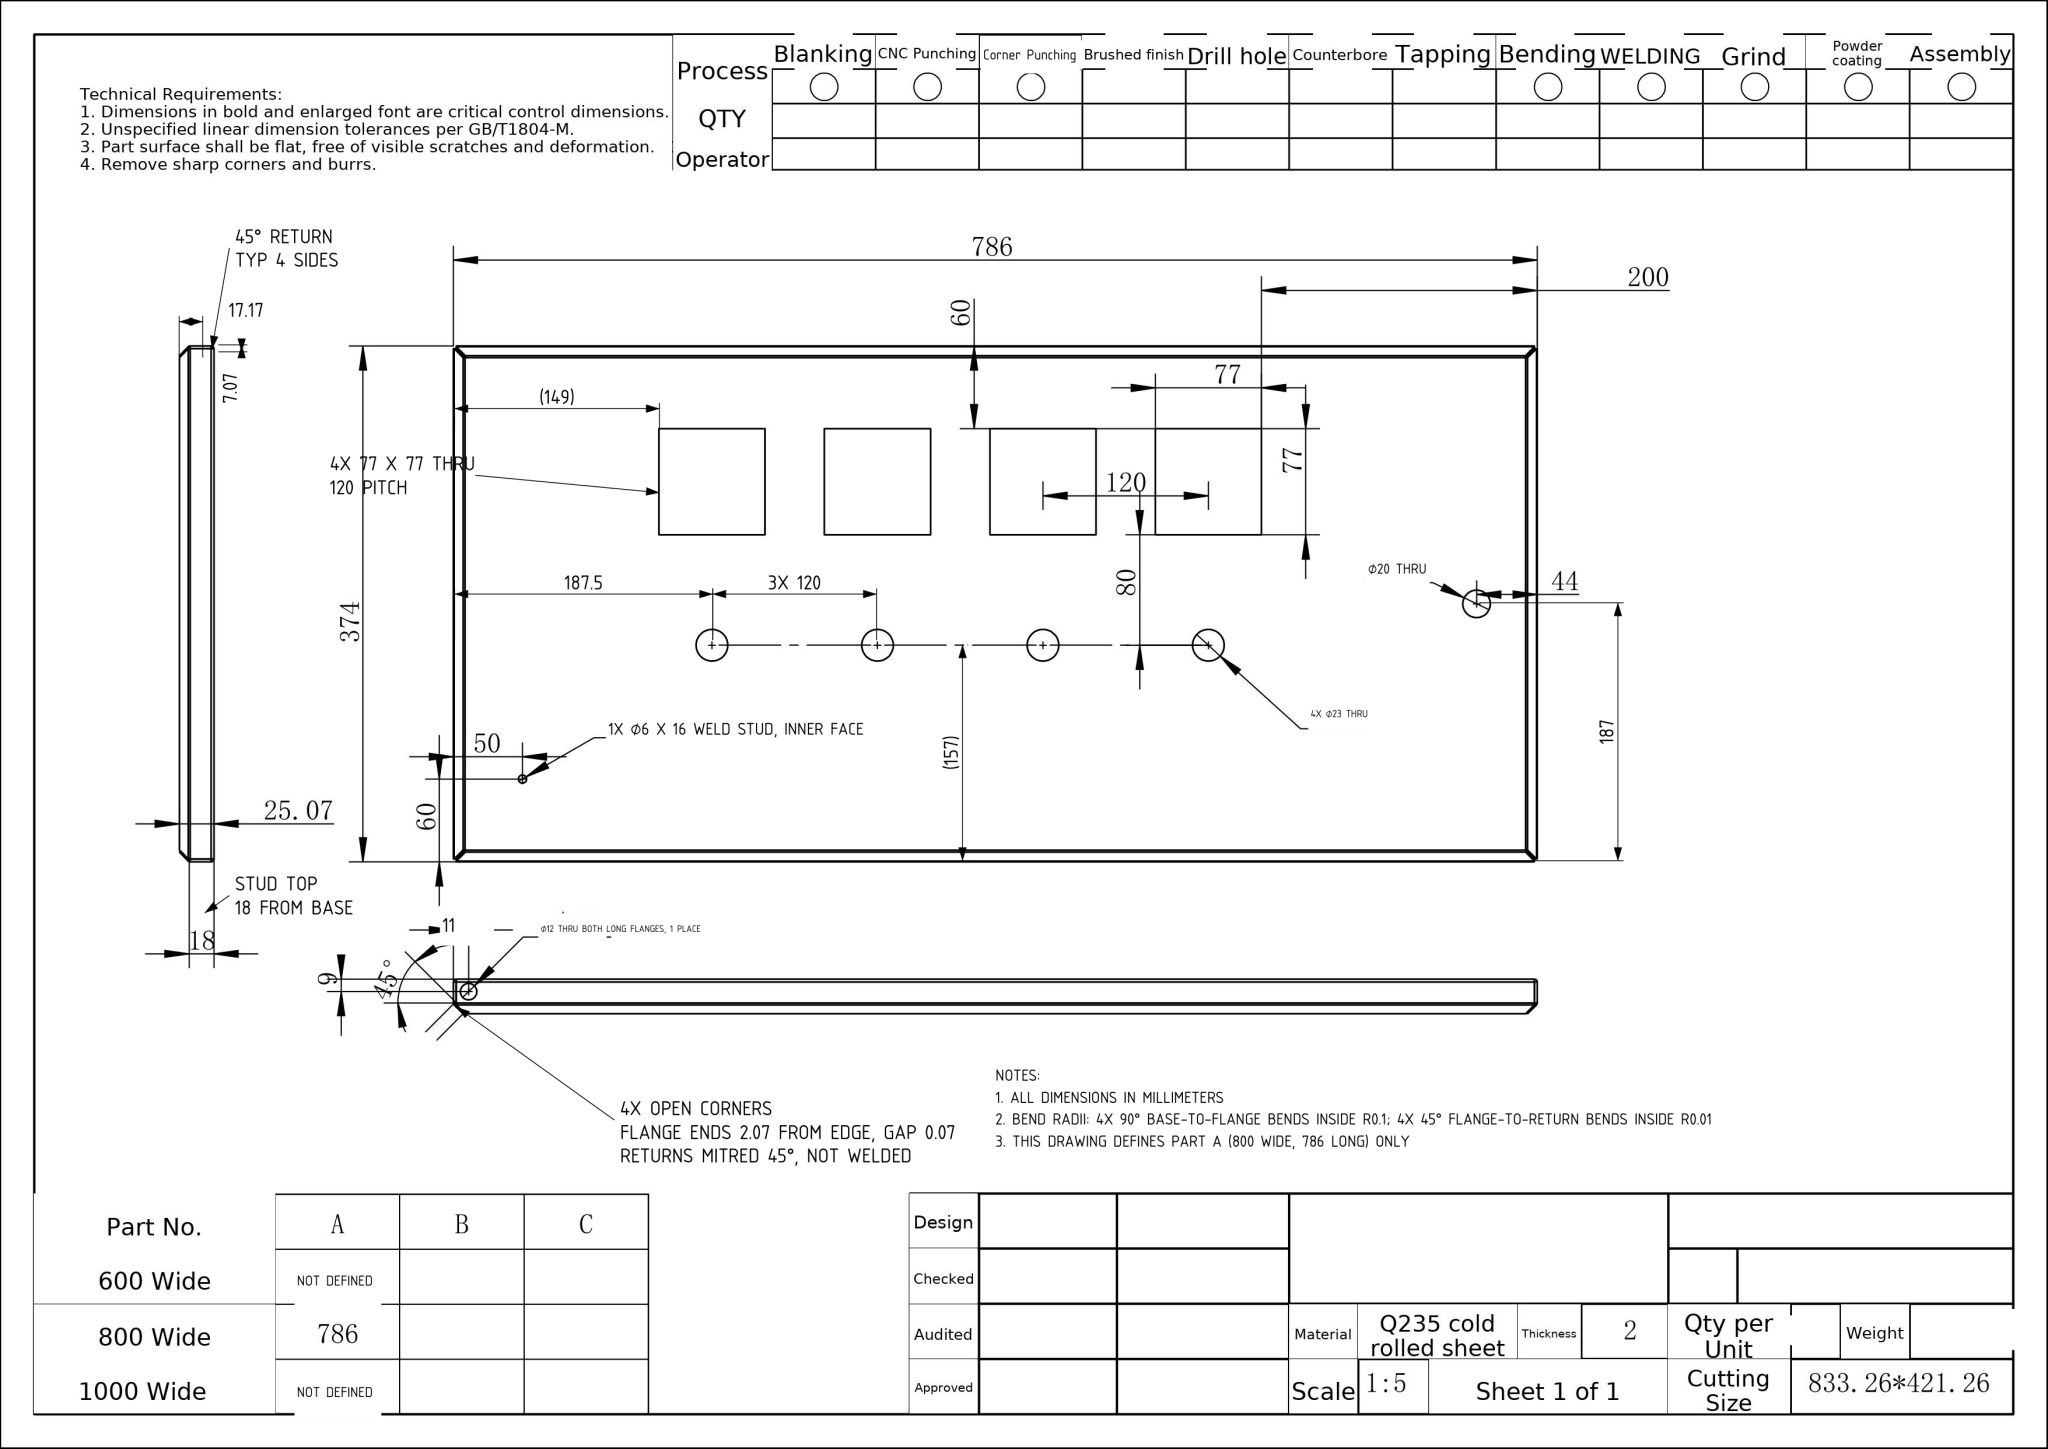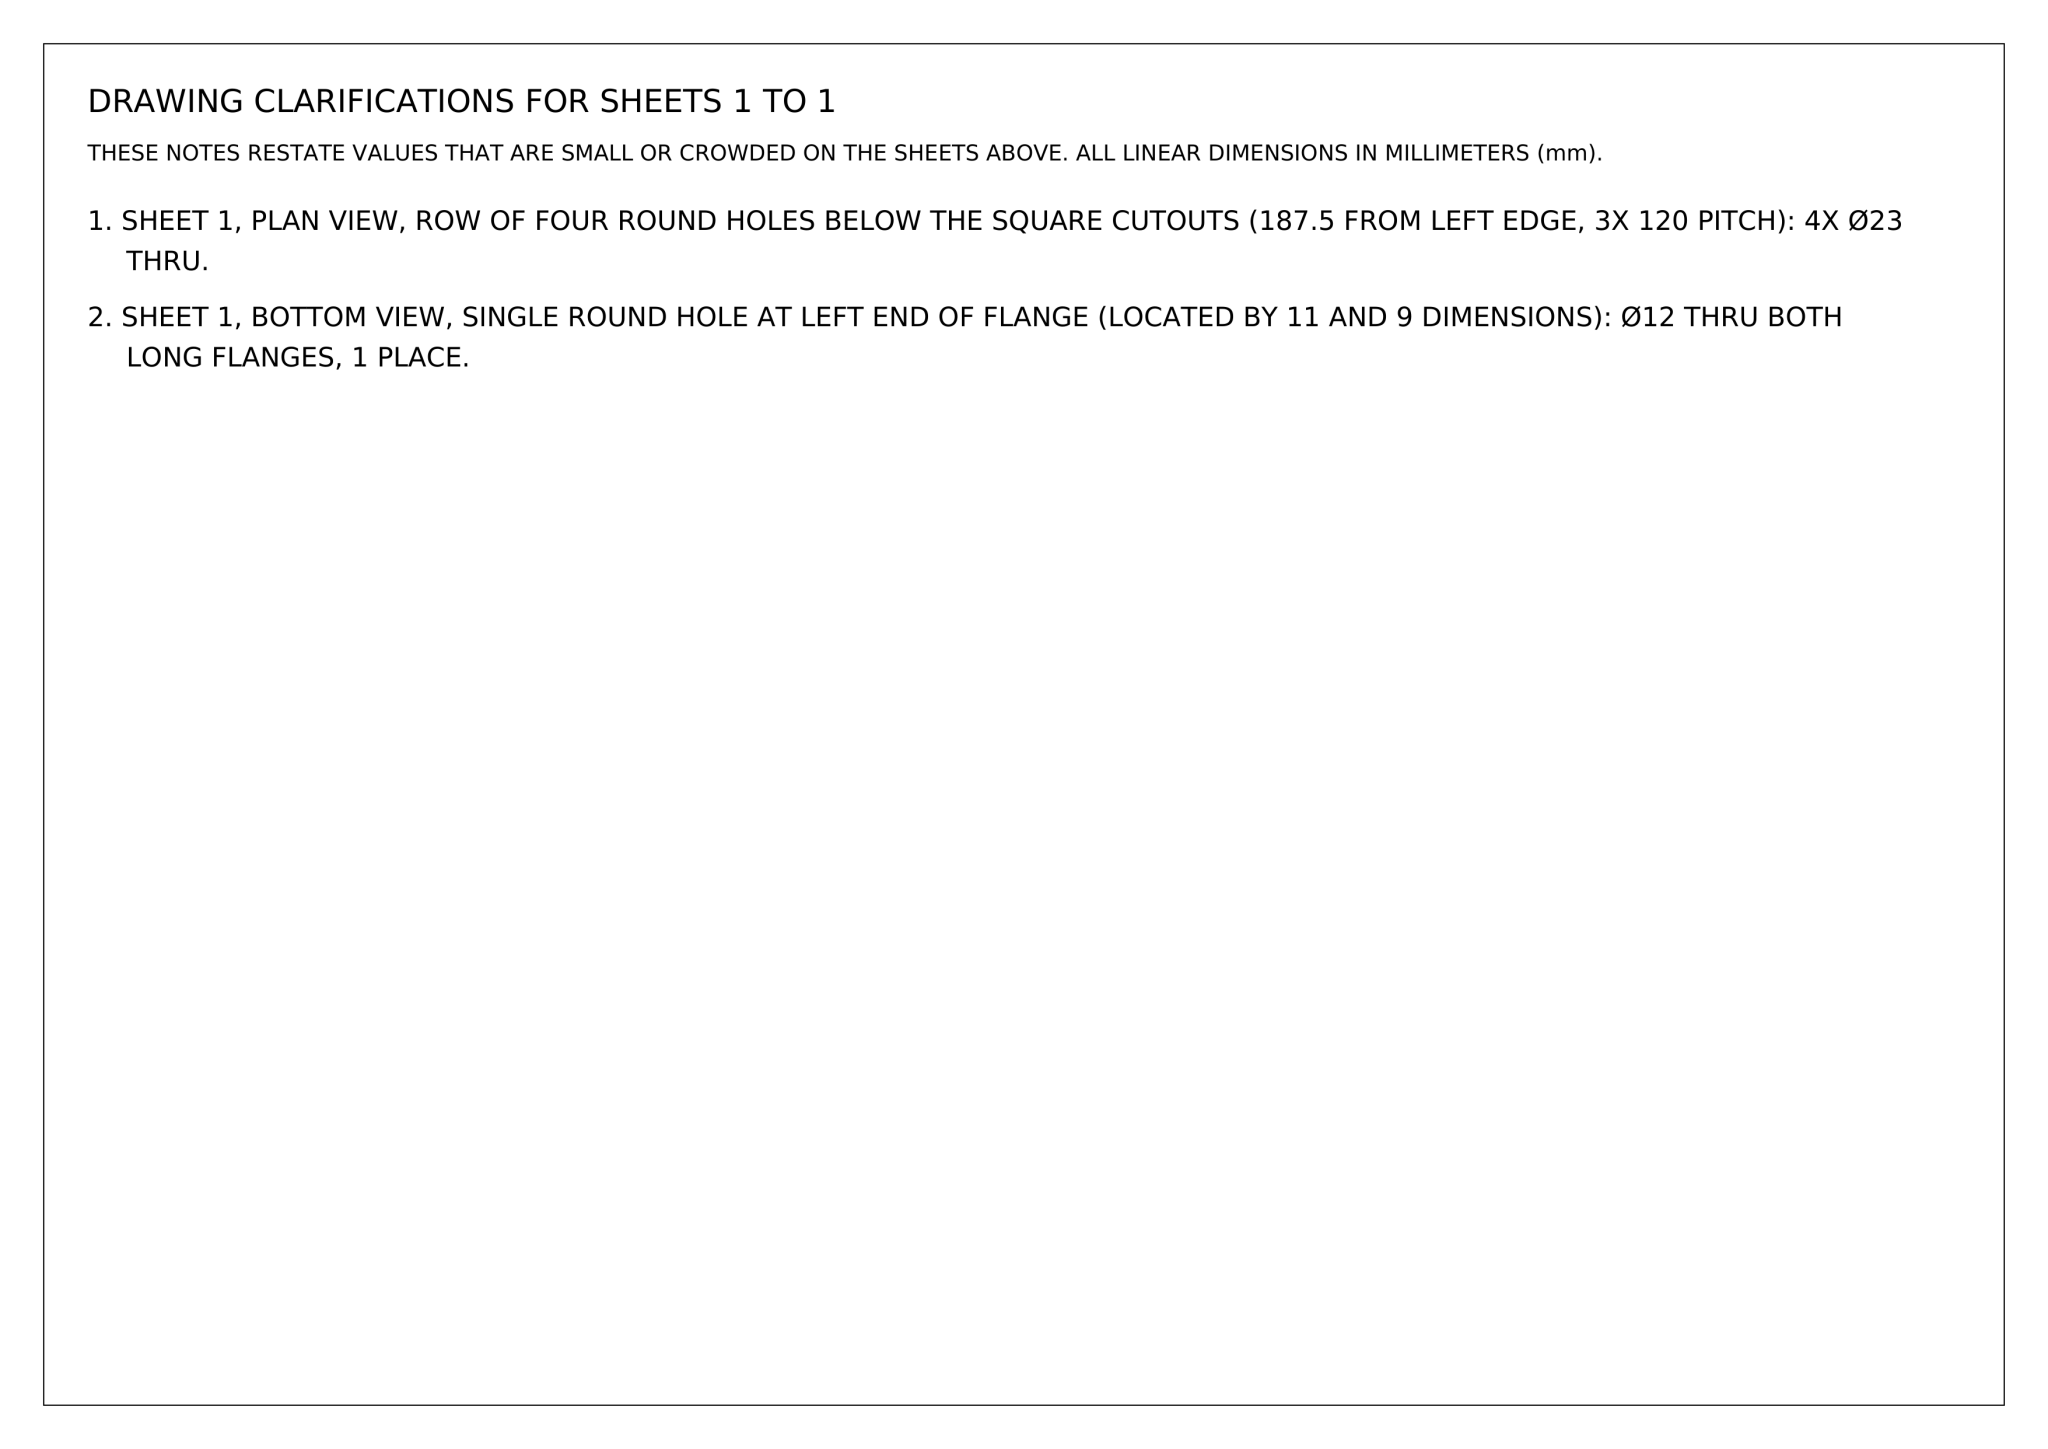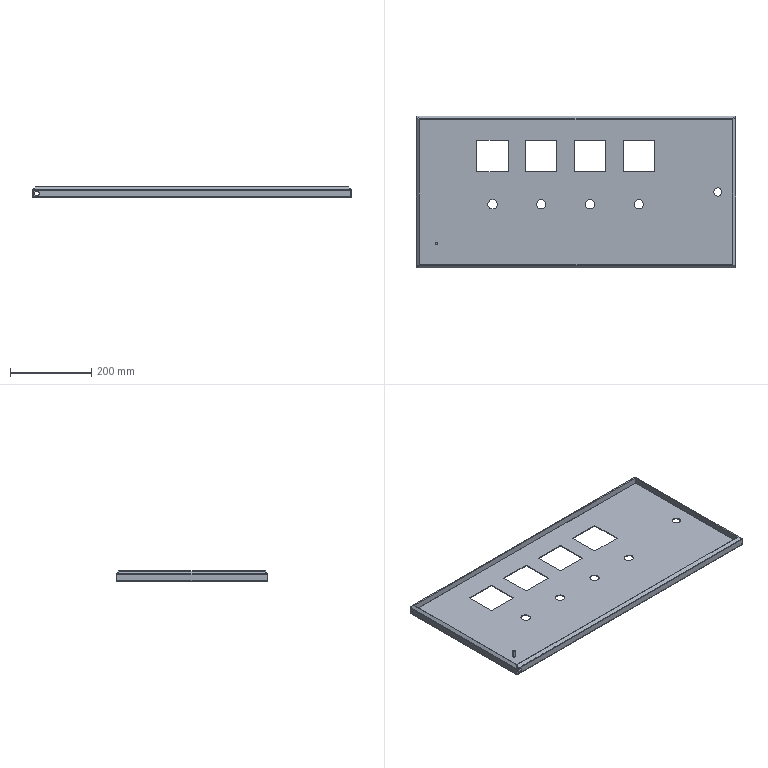Part | NX | mm | 1 solid | 103 faces | box 786 x 374 x 25.07 mm | volume 649620 mm3 | plane 55 | cylinder 32 | spline 16 | commonest cylinder face diameters 23 x8 12 x4 4.2 x4 0.2 x4 4.02 x4 0.02 x4 20 x2 6 x2